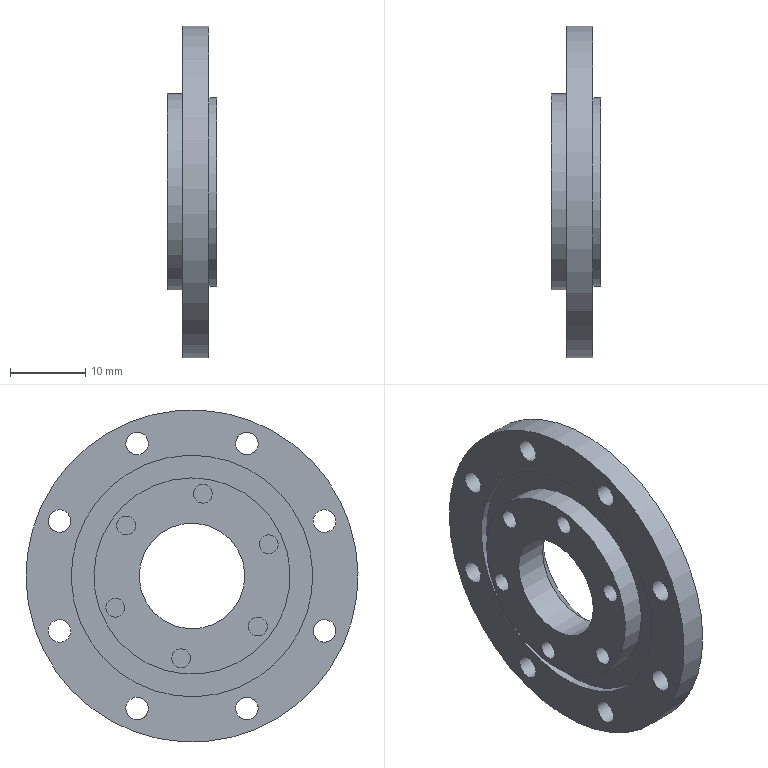Component | NX | END_CAP_2 | 1 solid | 31 faces | volume 5159 mm3 | cylinder 19 | plane 11 | cone 1 | commonest cylinder face diameters 3 x8 2.5 x6 25 x1 44 x1 26 x1 14 x1 32 x1